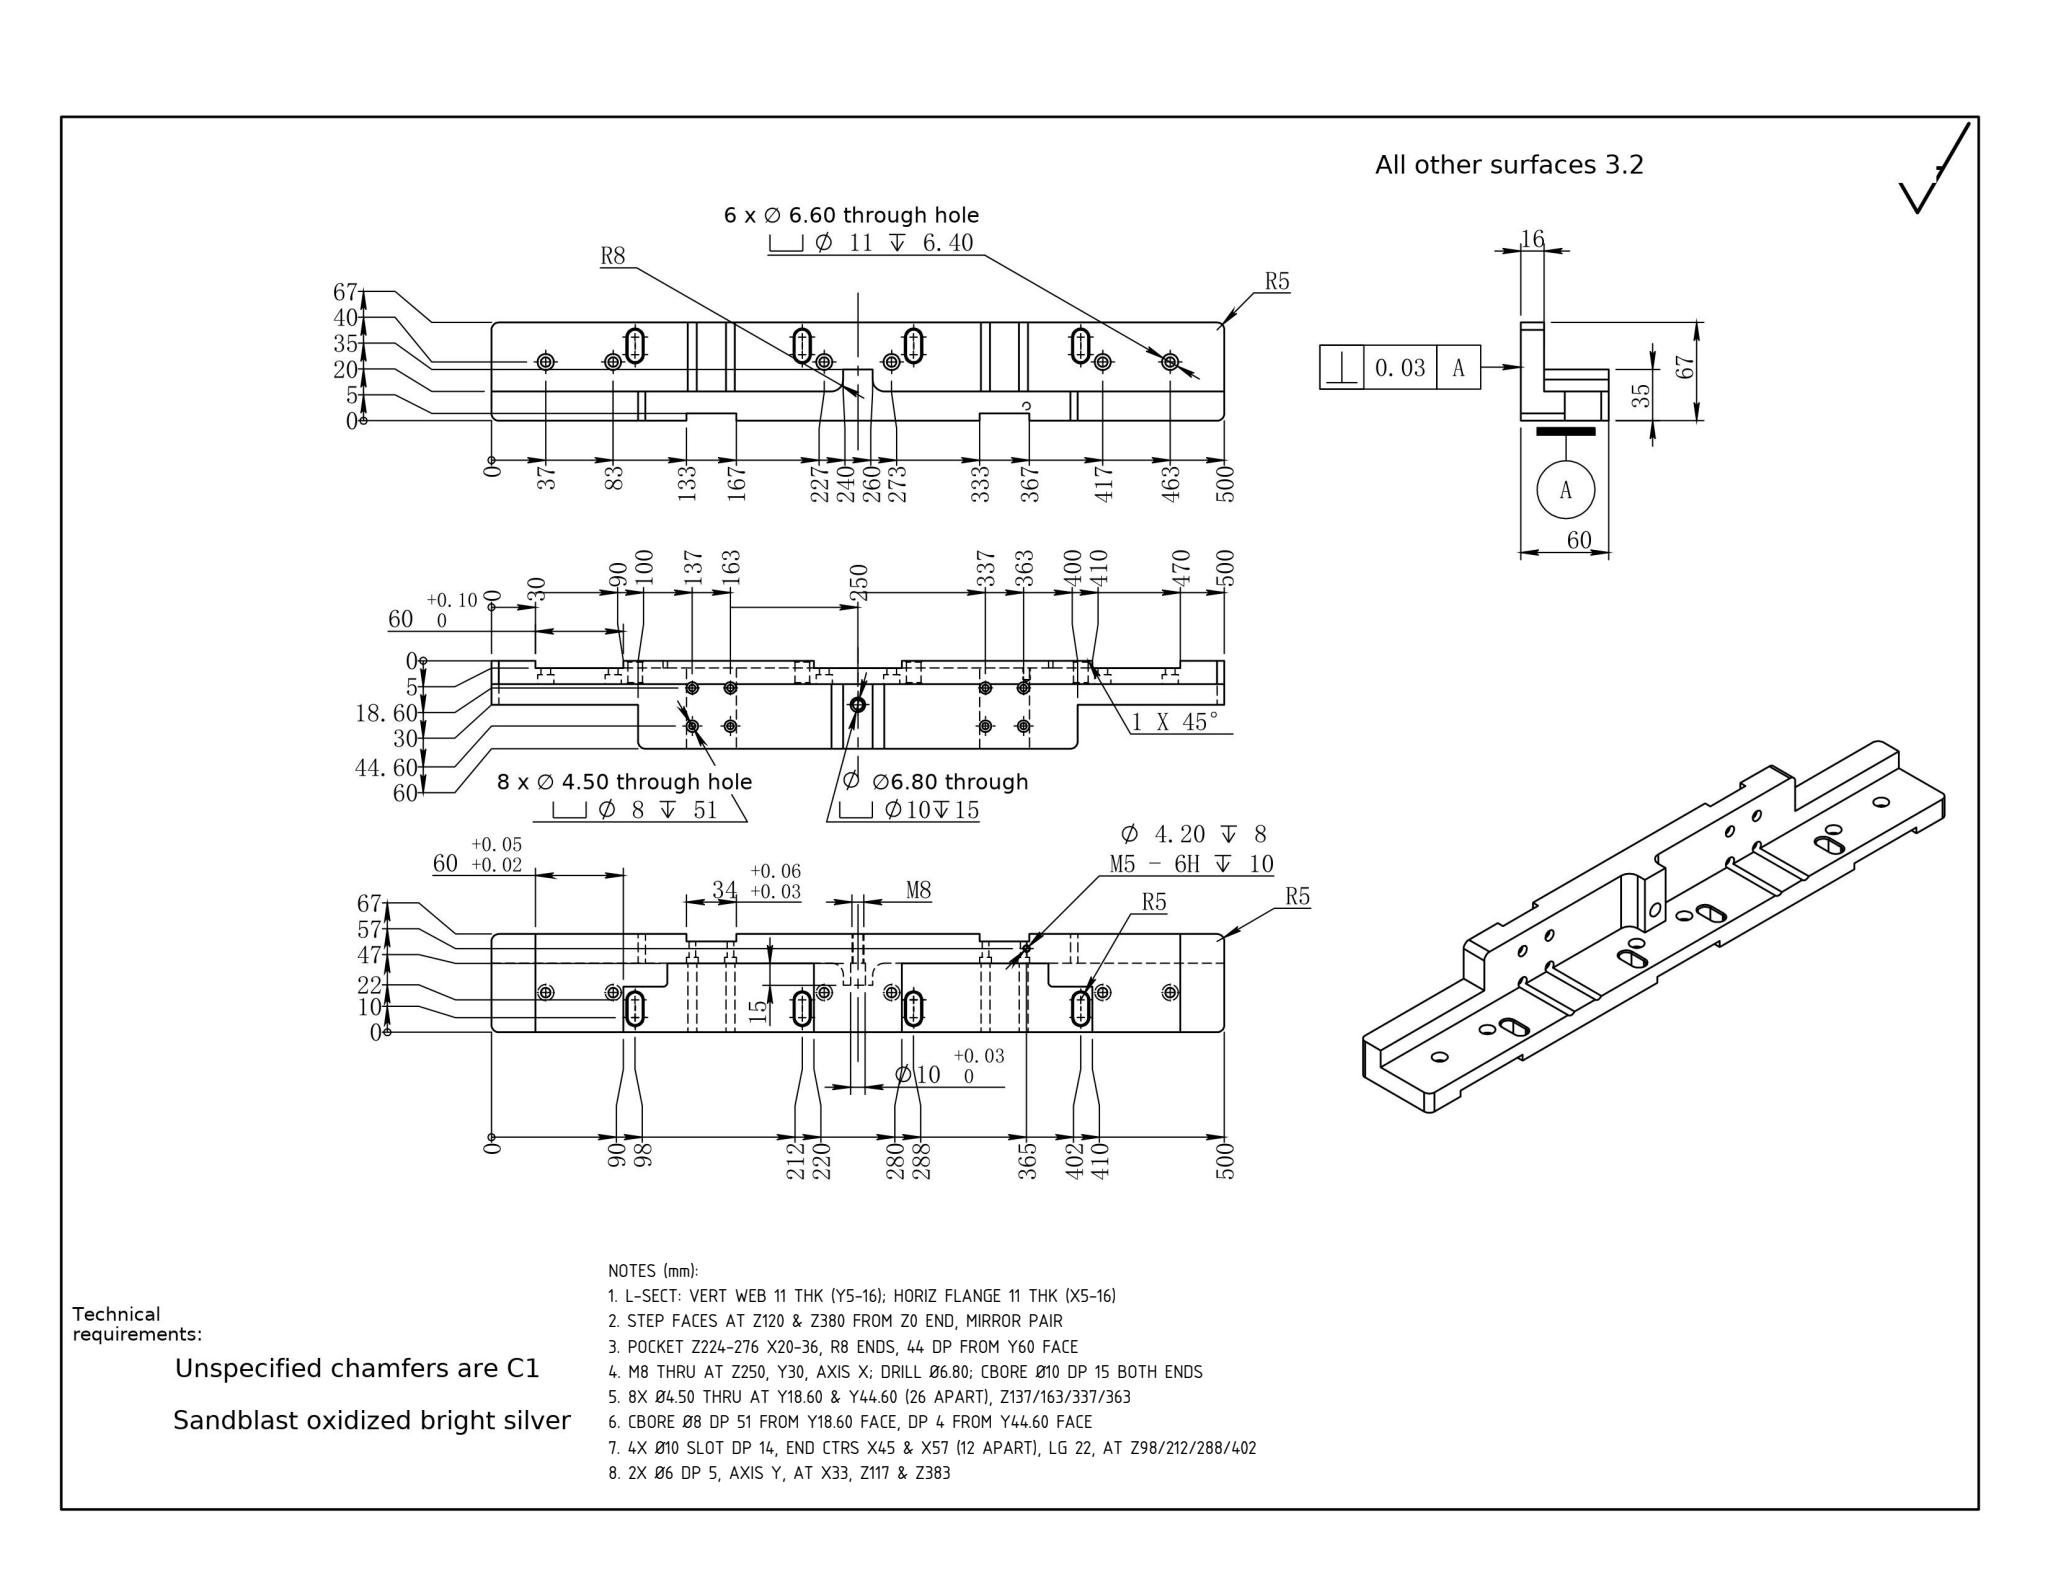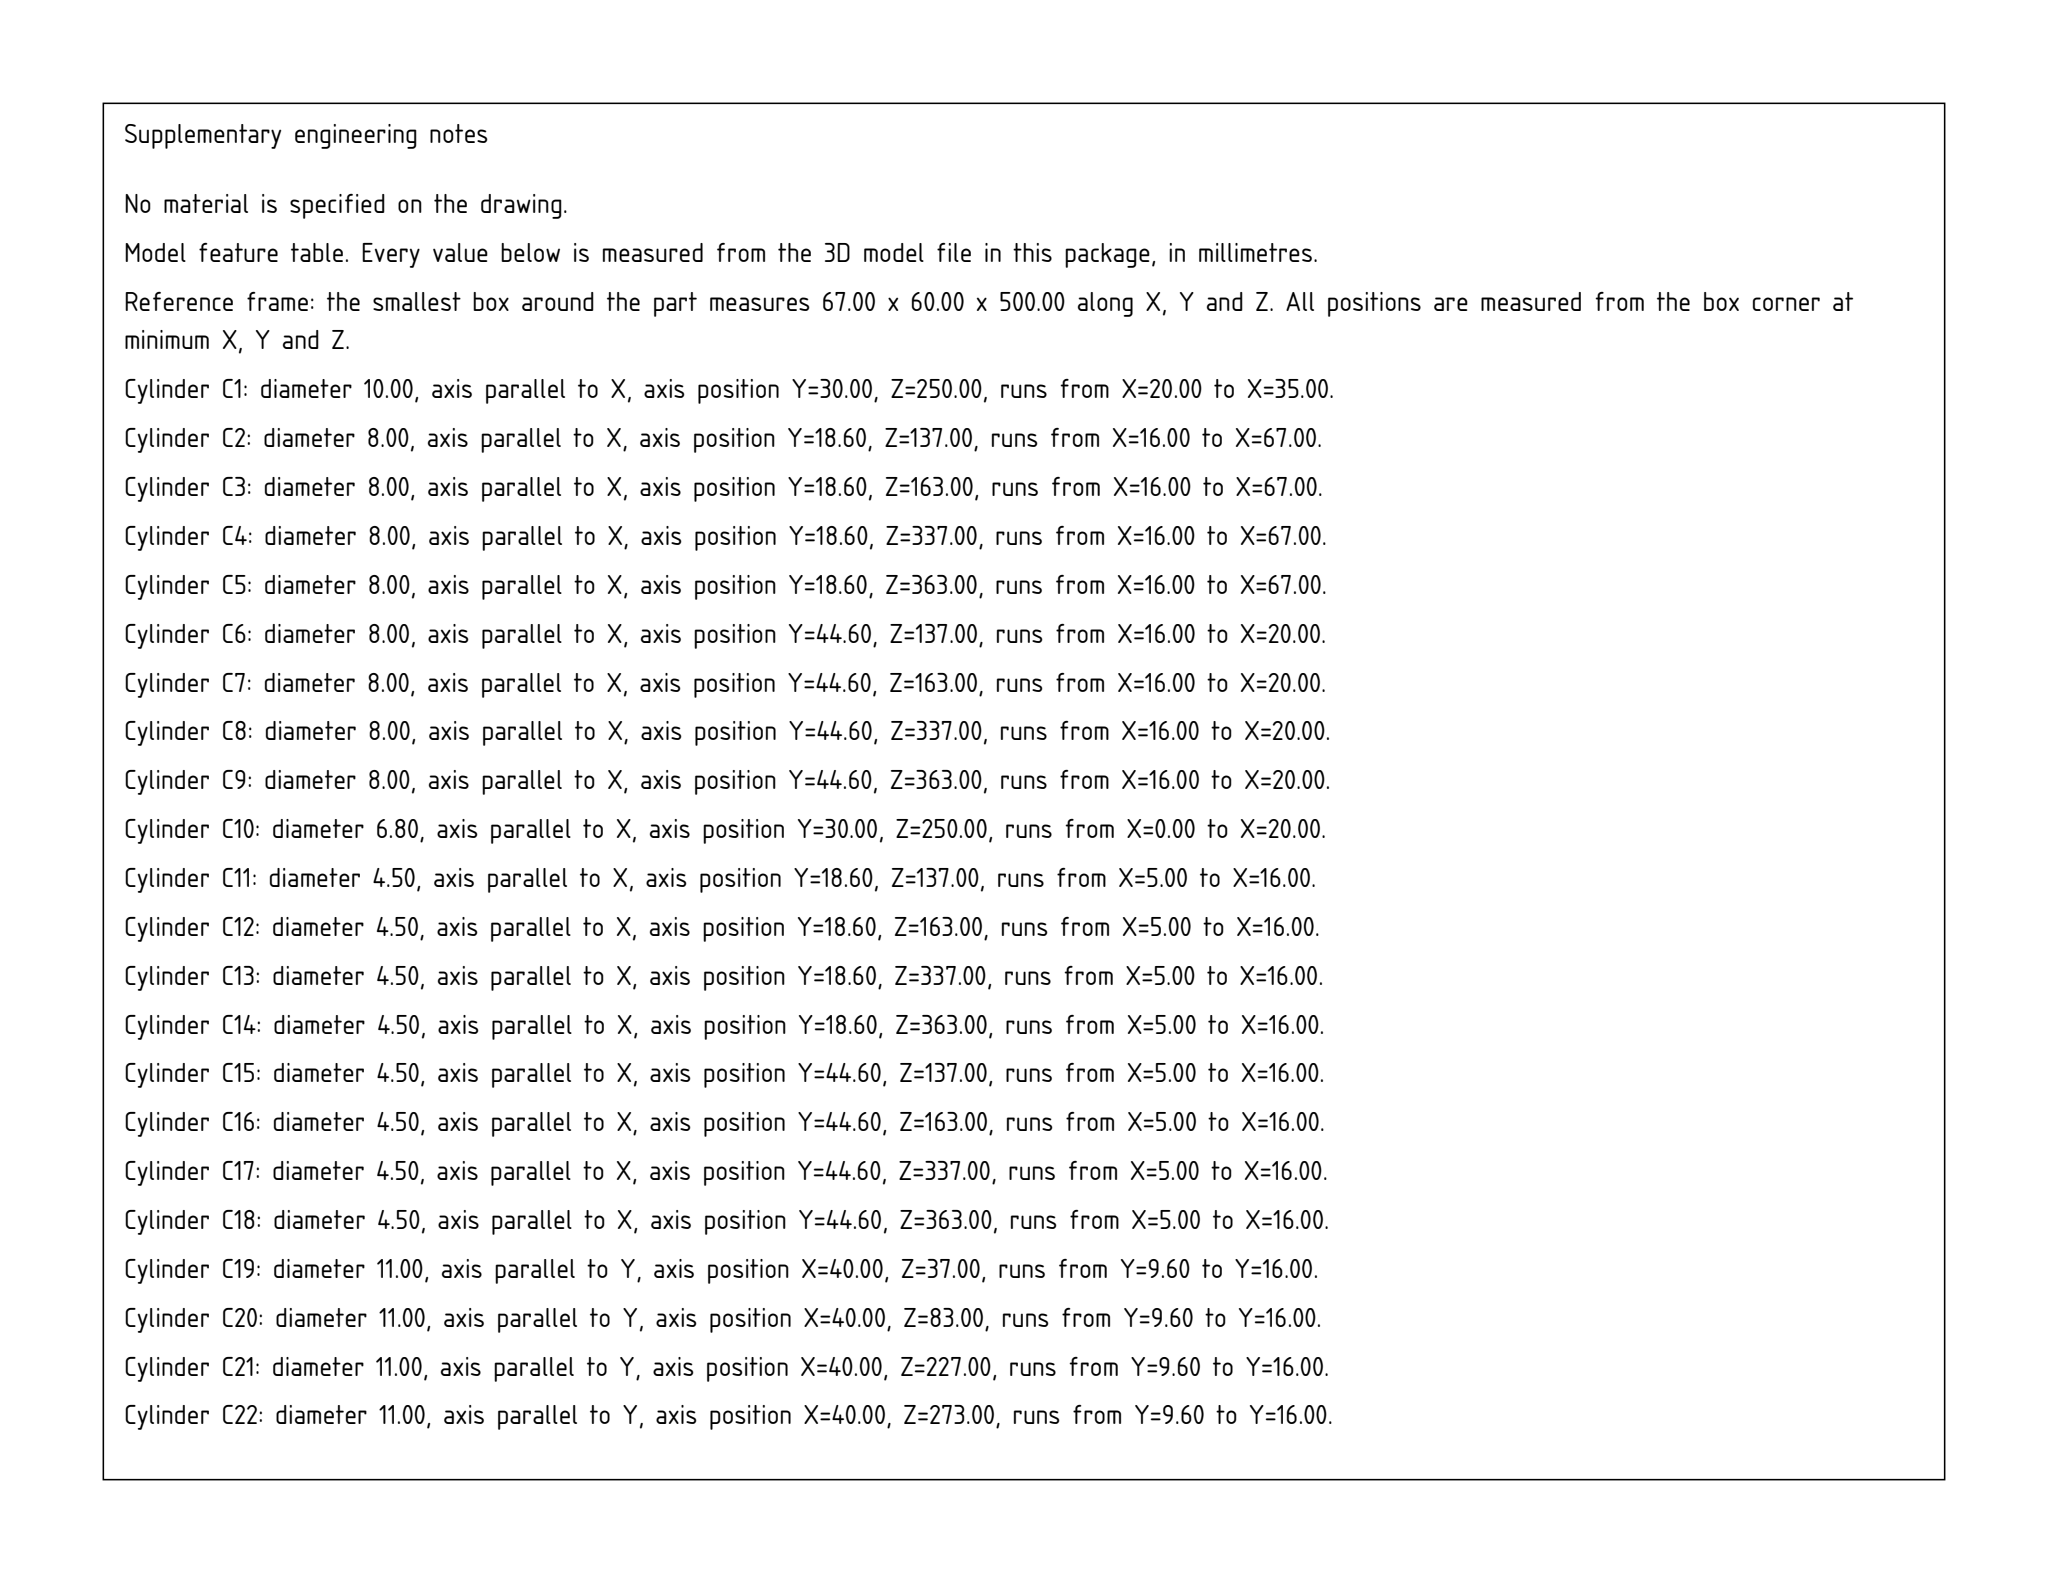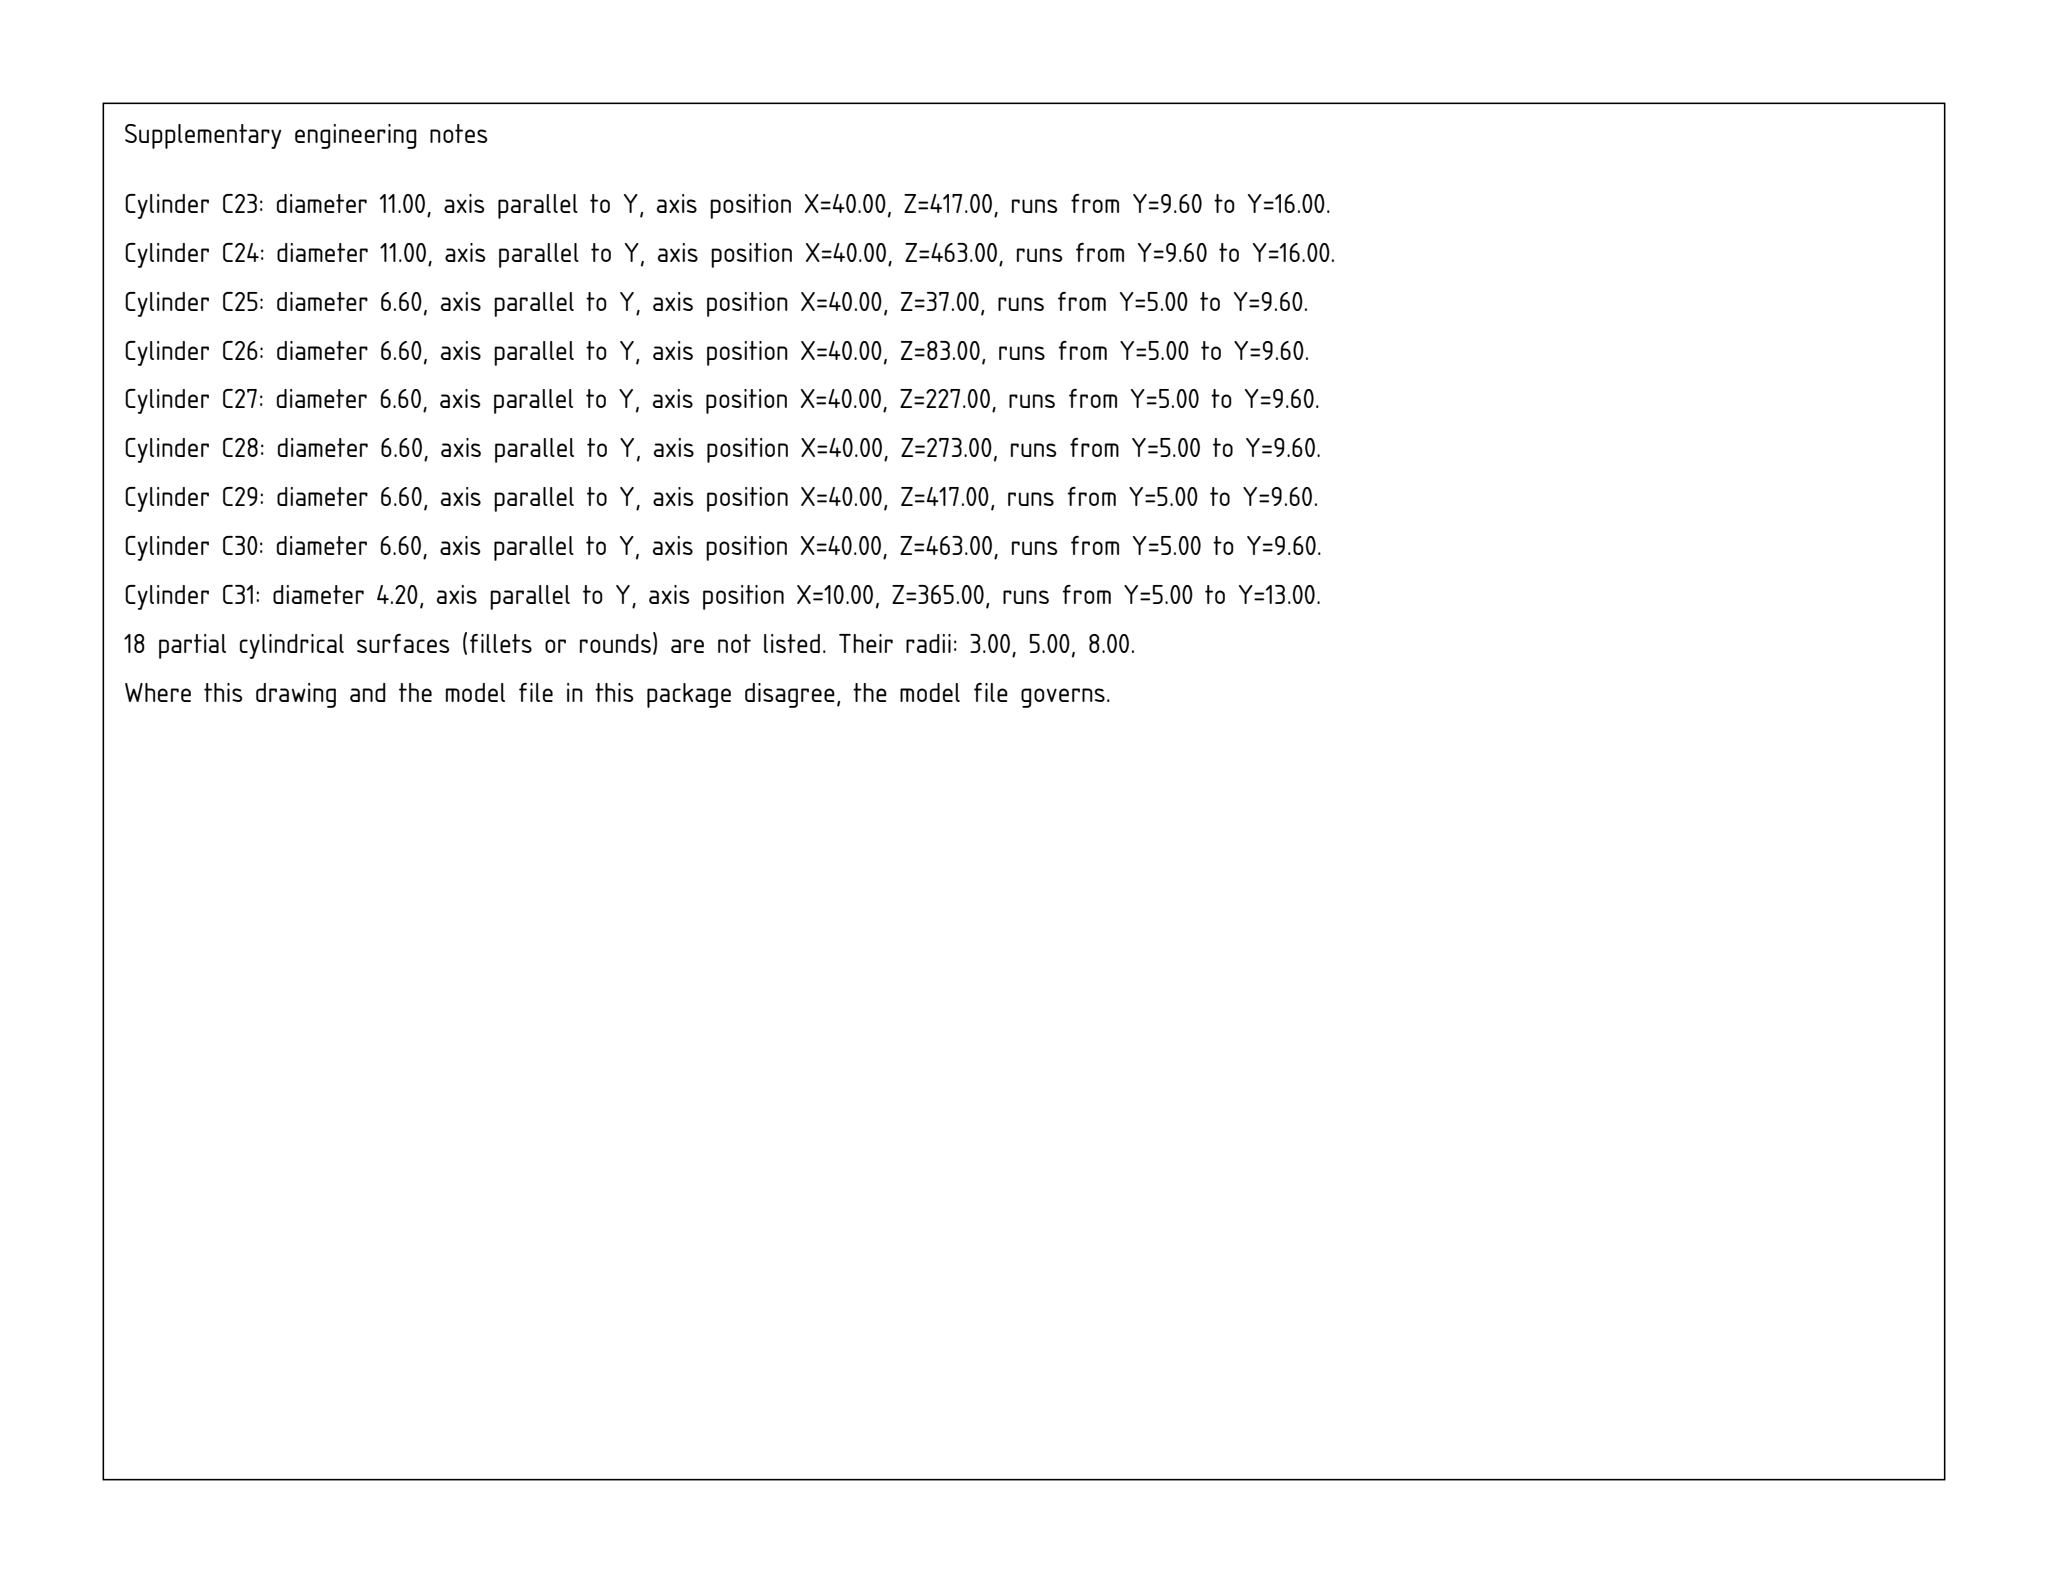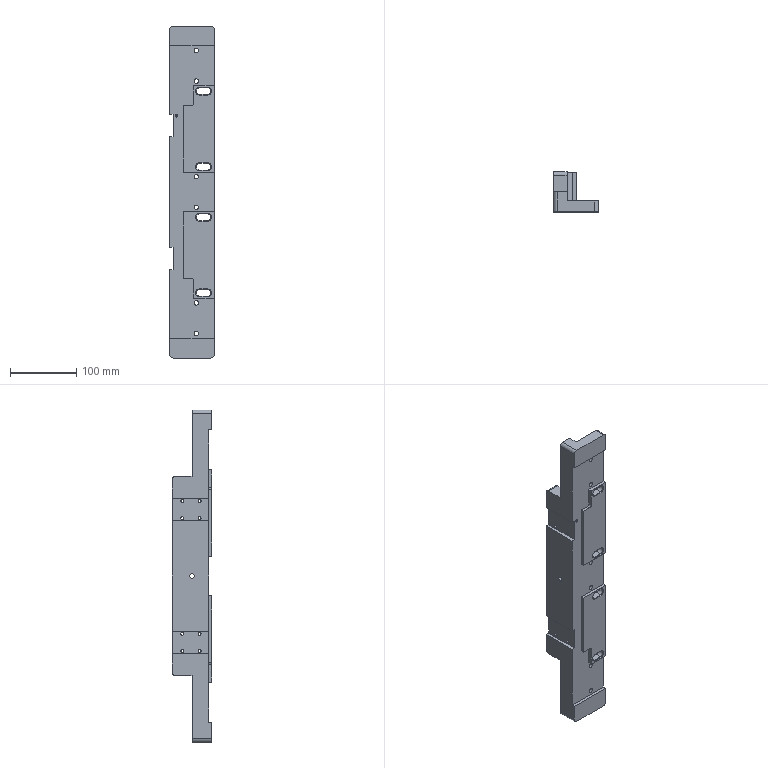Part | SolidWorks | mm | 1 solid | 181 faces | box 67 x 60 x 500 mm | volume 736250 mm3 | plane 83 | cylinder 80 | cone 18 | commonest cylinder face diameters 10 x16 4.5 x16 8 x16 11 x12 6.6 x12 4.2 x2 6.8 x2 16 x2
Drawing notes:
L-SECT: VERT WEB 11 THK (Y5-16); HORIZ FLANGE 11 THK (X5-16) | from the solid: y-planes 5 & 16 and x-planes 5 & 16; Ø6.6 len 4.6 + Ø11 cbore 6.4 = 11 thru wall; Ø4.5 x-holes len 11 thru plate
STEP FACES AT Z120 & Z380 FROM Z0 END, MIRROR PAIR | from the solid: z-normal planes at 120.0 and 380.0
POCKET Z224-276 X20-36, R8 ENDS, 44 DP FROM Y60 FACE | from the solid: Ø16 y-axis cyls at x28, z232 & z268, len 44 (R8 ends); walls x20 & x36, z224-276
M8 THRU AT Z250, Y30, AXIS X; DRILL Ø6.80; CBORE Ø10 DP 15 BOTH ENDS | from the solid: Ø6.8 x-axis cyl at y30, z250, len 20 x2 (thru 67); Ø10 x-axis cbore same axis, len 15 x2
8X Ø4.50 THRU AT Y18.60 & Y44.60 (26 APART), Z137/163/337/363 | from the solid: Ø4.5 x-axis cyls len 11 at y18.6 & 44.6, z=137,163,337,363
CBORE Ø8 DP 51 FROM Y18.60 FACE, DP 4 FROM Y44.60 FACE | from the solid: Ø8 axis-x cbores len 51 & 4 at y18.6; len 4 at y44.6
4X Ø10 SLOT DP 14, END CTRS X45 & X57 (12 APART), LG 22, AT Z98/212/288/402 | from the solid: Ø10 axis-y cyls at x45 & x57 for z98,212,288,402, length 14
2X Ø6 DP 5, AXIS Y, AT X33, Z117 & Z383 | from the solid: Ø6 axis-y cyls at (x33,z117) & (x33,z383), length 5
build123d program:
from build123d import *

# Parameters (mm, degrees)
SKETCH1_W                                       = 67
SKETCH1_H                                       = 60
BOSS_EXTRUDE1_DEPTH                             = 250
SKETCH2_W                                       = 47
SKETCH2_H                                       = 44
CUT_EXTRUDE1_DEPTH                              = 503.018
SKETCH3_W                                       = 34
SKETCH3_H                                       = 60
CUT_EXTRUDE2_DEPTH                              = 5
SKETCH4_W                                       = 67
SKETCH4_H                                       = 60
CUT_EXTRUDE3_DEPTH                              = 5
SKETCH5_W                                       = 20
SKETCH5_H                                       = 440
CUT_EXTRUDE4_DEPTH                              = 259.161
SKETCH9_W                                       = 100
SKETCH9_H                                       = 30
CUT_EXTRUDE5_DEPTH                              = 257.143
M4_HEX_SOCKET_HEAD_CAP_SCREW_CBORE1_D           = 4.5
M4_HEX_SOCKET_HEAD_CAP_SCREW_CBORE1_CBORE_D     = 8
M4_HEX_SOCKET_HEAD_CAP_SCREW_CBORE1_CBORE_DEPTH = 51
M6_HEX_SOCKET_HEAD_CAP_SCREW_CBORE1_D           = 6.6
M6_HEX_SOCKET_HEAD_CAP_SCREW_CBORE1_CBORE_D     = 11
M6_HEX_SOCKET_HEAD_CAP_SCREW_CBORE1_CBORE_DEPTH = 6.4
LPATTERN1_COUNT                                 = 3
LPATTERN1_PITCH                                 = 190
SKETCH16_W                                      = 20
SKETCH16_H                                      = 44
BOSS_EXTRUDE2_DEPTH                             = 15
M8_TAPPED_HOLE1_D                               = 6.8
SKETCH15_R                                      = 5
CUT_EXTRUDE6_DEPTH                              = 15
FILLET1_R                                       = 8
FILLET2_R                                       = 5
FILLET3_R                                       = 5
M5_TAPPED_HOLE1_D                               = 4.2
M5_TAPPED_HOLE1_DEPTH                           = 8
M5_TAPPED_HOLE1_TIP                             = 1.262
CUT_EXTRUDE7_DEPTH                              = 260.273
CHAMFER1_SIZE                                   = 1
SKETCH21_W                                      = 16
SKETCH21_H                                      = 30
CUT_EXTRUDE8_DEPTH                              = 259.161
FILLET4_R                                       = 3


with BuildPart() as part:
    # Sketch1 → Boss-Extrude1 (new, symmetric)
    with BuildSketch(Plane.XY):
        Rectangle(SKETCH1_W, SKETCH1_H)
    extrude(amount=BOSS_EXTRUDE1_DEPTH, both=True)

    # Sketch2 → Cut-Extrude1 (cut, through all)
    with BuildSketch(Plane.XY.offset(250)):
        with Locations((10, 8)):
            Rectangle(SKETCH2_W, SKETCH2_H)
    extrude(amount=-CUT_EXTRUDE1_DEPTH, mode=Mode.SUBTRACT)

    # Sketch3 → Cut-Extrude2 (cut)
    with BuildSketch(Plane.ZY.offset(33.5)):
        with Locations((-100, 0)):
            Rectangle(SKETCH3_W, SKETCH3_H)
        with Locations((100, 0)):
            Rectangle(SKETCH3_W, SKETCH3_H)
    extrude(amount=-CUT_EXTRUDE2_DEPTH, mode=Mode.SUBTRACT)

    # Sketch4 → Cut-Extrude3 (cut)
    with BuildSketch(Plane.XZ.offset(30)):
        Rectangle(SKETCH4_W, SKETCH4_H)
        with Locations((0, 190)):
            Rectangle(SKETCH4_W, SKETCH4_H)
        with Locations((0, -190)):
            Rectangle(SKETCH4_W, SKETCH4_H)
    extrude(amount=-CUT_EXTRUDE3_DEPTH, mode=Mode.SUBTRACT)

    # Sketch5 → Cut-Extrude4 (cut, through all)
    with BuildSketch(Plane.XZ.offset(25)):
        with Locations((-23.5, 0)):
            Rectangle(SKETCH5_W, SKETCH5_H)
    extrude(amount=CUT_EXTRUDE4_DEPTH, mode=Mode.SUBTRACT)

    # Sketch9 → Cut-Extrude5 (cut, through all)
    with BuildSketch(Plane(origin=(-13.5, 0, 0), x_dir=(0, 0, -1), z_dir=(1, 0, 0))):
        with Locations((-200, 15)):
            Rectangle(SKETCH9_W, SKETCH9_H)
    cut_extrude5 = extrude(amount=-CUT_EXTRUDE5_DEPTH, mode=Mode.SUBTRACT)

    # Mirror1: Cut-Extrude5 across plane
    add(cut_extrude5.mirror(Plane.XY), mode=Mode.SUBTRACT)

    # M4 Hex Socket Head Cap Screw CBORE1 (through all)
    with Locations(Plane(origin=(33.5, 0, 0), x_dir=(0, 0, -1), z_dir=(1, 0, 0))):
        with Locations((-113, 14.6), (-113, -11.4), (-87, 14.6), (-87, -11.4)):
            m4_hex_socket_head_cap_screw_cbore1 = CounterBoreHole(M4_HEX_SOCKET_HEAD_CAP_SCREW_CBORE1_D / 2, M4_HEX_SOCKET_HEAD_CAP_SCREW_CBORE1_CBORE_D / 2, M4_HEX_SOCKET_HEAD_CAP_SCREW_CBORE1_CBORE_DEPTH)

    # Mirror2: M4 Hex Socket Head Cap Screw CBORE1 across plane
    add(m4_hex_socket_head_cap_screw_cbore1.mirror(Plane.XY), mode=Mode.SUBTRACT)

    # M6 Hex Socket Head Cap Screw CBORE1 (through all)
    with Locations(Plane(origin=(0, -14, 0), x_dir=(1, 0, 0), z_dir=(0, 1, 0))):
        with Locations((6.5, 167), (6.5, 213)):
            m6_hex_socket_head_cap_screw_cbore1 = CounterBoreHole(M6_HEX_SOCKET_HEAD_CAP_SCREW_CBORE1_D / 2, M6_HEX_SOCKET_HEAD_CAP_SCREW_CBORE1_CBORE_D / 2, M6_HEX_SOCKET_HEAD_CAP_SCREW_CBORE1_CBORE_DEPTH)

    # LPattern1: M6 Hex Socket Head Cap Screw CBORE1 ×3
    with Locations(*[(0, 0, i * LPATTERN1_PITCH) for i in range(1, LPATTERN1_COUNT)]):
        add(m6_hex_socket_head_cap_screw_cbore1, mode=Mode.SUBTRACT)

    # Sketch16 → Boss-Extrude2 (add)
    with BuildSketch(Plane(origin=(-13.5, 0, 0), x_dir=(0, 0, -1), z_dir=(1, 0, 0))):
        with Locations((0, 8)):
            Rectangle(SKETCH16_W, SKETCH16_H)
    extrude(amount=BOSS_EXTRUDE2_DEPTH)

    # M8 Tapped Hole1 (through all)
    with Locations(Plane(origin=(1.5, 0, 0), x_dir=(0, 0, -1), z_dir=(1, 0, 0))):
        with Locations((0, 0)):
            Hole(M8_TAPPED_HOLE1_D / 2)

    # Sketch15 → Cut-Extrude6 (cut)
    with BuildSketch(Plane(origin=(1.5, 0, 0), x_dir=(0, 0, -1), z_dir=(1, 0, 0))):
        with Locations(Location((0, 0, 0), (0, 0, 90))):
            Circle(SKETCH15_R)
    extrude(amount=-CUT_EXTRUDE6_DEPTH, mode=Mode.SUBTRACT)

    # Fillet1
    fillet1_edges = [part.edges().sort_by_distance(p)[0] for p in [
        (-13.5, 8, -10),
        (-13.5, 8, 10),
    ]]
    fillet(fillet1_edges, radius=FILLET1_R)

    # Fillet2
    fillet2_edges = [part.edges().sort_by_distance(p)[0] for p in [
        (-33.5, -15, 250),
        (-33.5, -15, -250),
        (33.5, -22, 250),
        (33.5, -22, -250),
    ]]
    fillet(fillet2_edges, radius=FILLET2_R)

    # Fillet3
    fillet3_edges = [part.edges().sort_by_distance(p)[0] for p in [
        (-23.5, 30, 150),
        (-23.5, 30, -150),
    ]]
    fillet(fillet3_edges, radius=FILLET3_R)

    # M5 Tapped Hole1
    with Locations(Plane(origin=(0, -25, 0), x_dir=(-1, 0, 0), z_dir=(0, -1, 0))):
        with Locations((23.5, -115)):
            Hole(M5_TAPPED_HOLE1_D / 2, depth=M5_TAPPED_HOLE1_DEPTH)
            with Locations((0, 0, -(M5_TAPPED_HOLE1_DEPTH + M5_TAPPED_HOLE1_TIP / 2))):  # 118° drill point
                Cone(0, M5_TAPPED_HOLE1_D / 2, M5_TAPPED_HOLE1_TIP, mode=Mode.SUBTRACT)

    # Sketch20 → Cut-Extrude7 (cut, through all)
    with BuildSketch(Plane.XZ.offset(30)):
        with BuildLine():
            Line((11.5, -147), (23.5, -147))
            ThreePointArc((23.5, -147), (28.5, -152), (23.5, -157))
            Line((23.5, -157), (11.5, -157))
            ThreePointArc((11.5, -157), (6.5, -152), (11.5, -147))
        make_face()
        with BuildLine():
            Line((23.5, 33), (11.5, 33))
            ThreePointArc((11.5, 33), (6.5, 38), (11.5, 43))
            Line((11.5, 43), (23.5, 43))
            ThreePointArc((23.5, 43), (28.5, 38), (23.5, 33))
        make_face()
        with BuildLine():
            Line((23.5, 147), (11.5, 147))
            ThreePointArc((11.5, 147), (6.5, 152), (11.5, 157))
            Line((11.5, 157), (23.5, 157))
            ThreePointArc((23.5, 157), (28.5, 152), (23.5, 147))
        make_face()
        with BuildLine():
            Line((11.5, -33), (23.5, -33))
            ThreePointArc((23.5, -33), (28.5, -38), (23.5, -43))
            Line((23.5, -43), (11.5, -43))
            ThreePointArc((11.5, -43), (6.5, -38), (11.5, -33))
        make_face()
    extrude(amount=-CUT_EXTRUDE7_DEPTH, mode=Mode.SUBTRACT)

    # Chamfer1
    chamfer1_edges = [part.edges().sort_by_distance(p)[0] for p in [
        (17.5, -14, 157),
        (6.5, -14, 152),
        (17.5, -14, 147),
        (28.5, -14, 152),
        (6.5, -14, -152),
        (17.5, -14, -147),
        (28.5, -14, -152),
        (17.5, -14, -157),
        (6.5, -30, -152),
        (17.5, -30, -157),
        (28.5, -30, -152),
        (17.5, -30, -147),
        (28.5, -14, 38),
        (17.5, -14, 33),
        (6.5, -14, 38),
        (17.5, -14, 43),
        (28.5, -30, 38),
        (17.5, -30, 43),
        (6.5, -30, 38),
        (17.5, -30, 33),
        (28.5, -30, 152),
        (17.5, -30, 157),
        (6.5, -30, 152),
        (17.5, -30, 147),
        (6.5, -14, -38),
        (17.5, -14, -33),
        (28.5, -14, -38),
        (17.5, -14, -43),
        (6.5, -30, -38),
        (17.5, -30, -43),
        (28.5, -30, -38),
        (17.5, -30, -33),
    ]]
    chamfer(chamfer1_edges, length=CHAMFER1_SIZE)

    # Sketch21 → Cut-Extrude8 (cut, through all)
    with BuildSketch(Plane.XZ.offset(25)):
        with Locations((-5.5, -145)):
            Rectangle(SKETCH21_W, SKETCH21_H)
        with Locations((-5.5, 145)):
            Rectangle(SKETCH21_W, SKETCH21_H)
    extrude(amount=CUT_EXTRUDE8_DEPTH, mode=Mode.SUBTRACT)

    # Fillet4
    fillet4_edges = [part.edges().sort_by_distance(p)[0] for p in [
        (2.5, -27.5, -130),
        (2.5, -27.5, 130),
    ]]
    fillet(fillet4_edges, radius=FILLET4_R)


solid = part.part